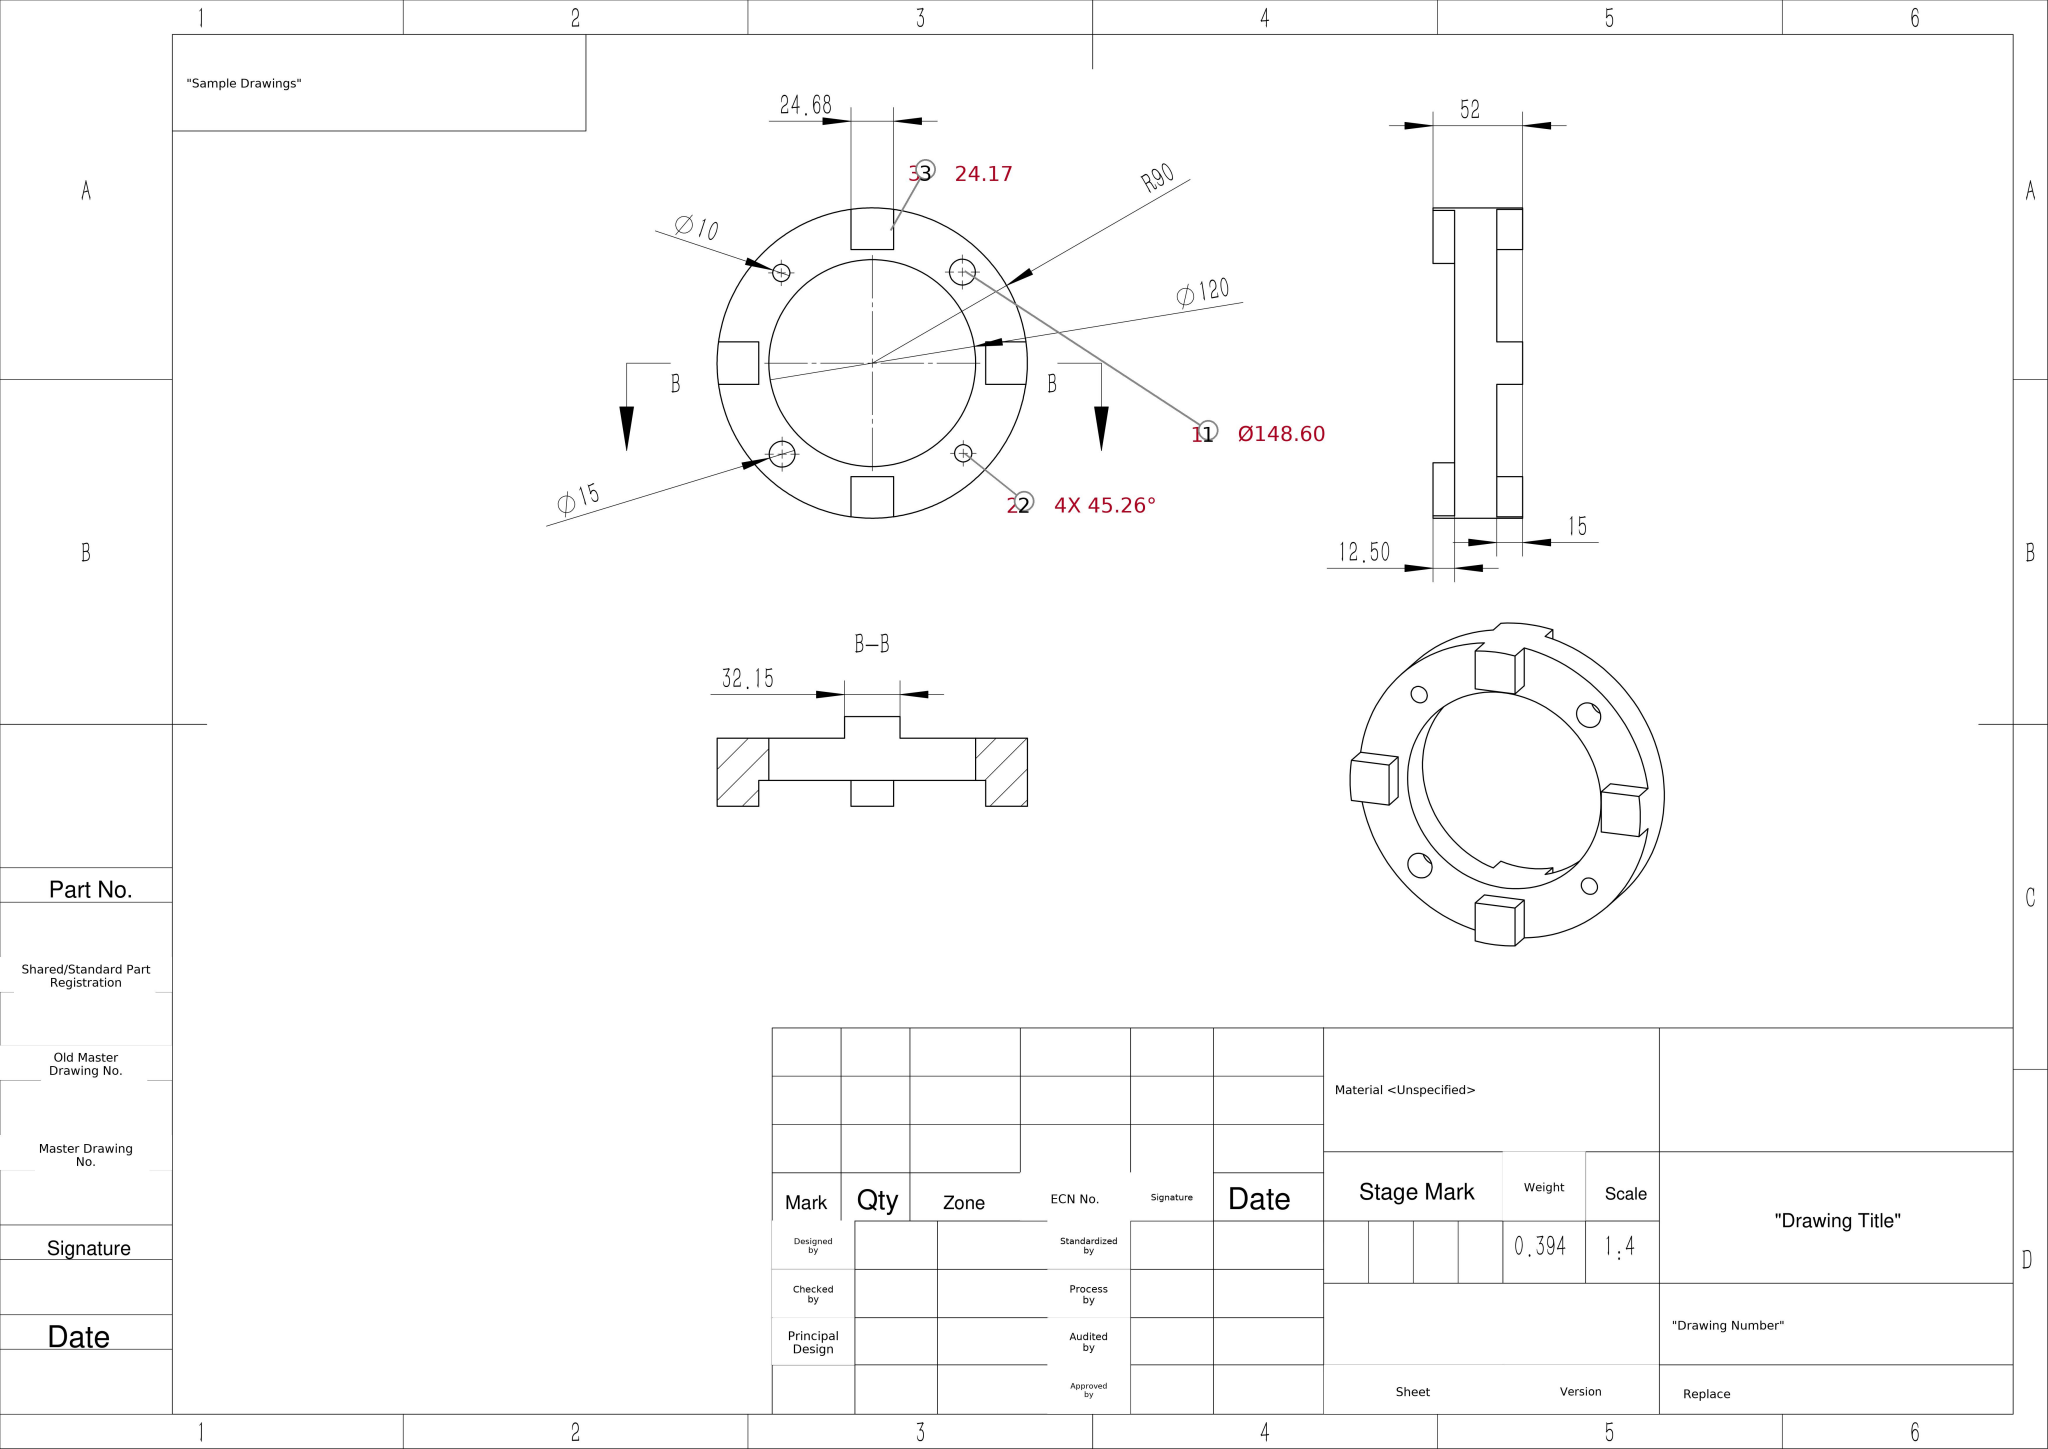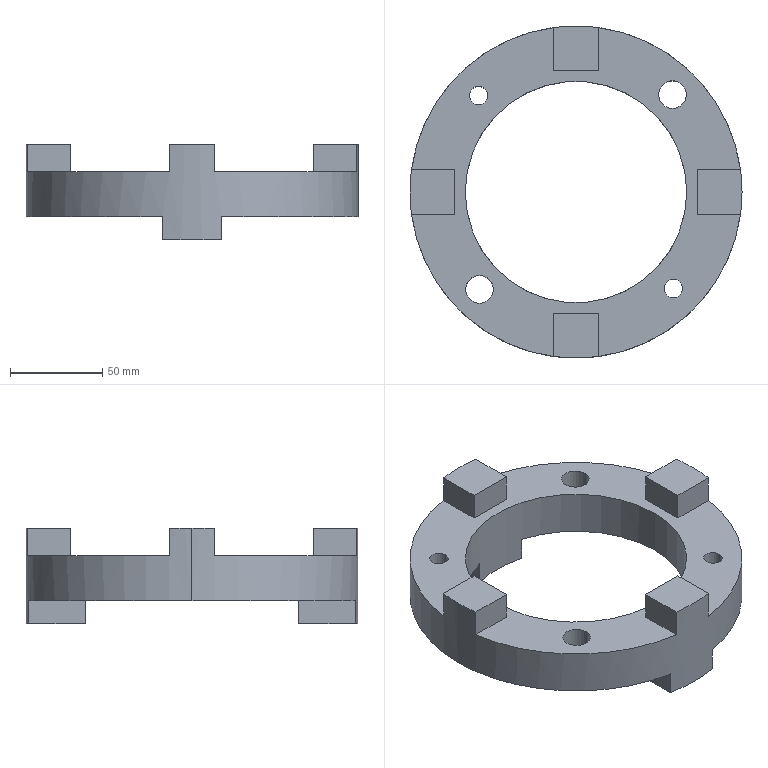Part | SolidWorks | mm | 1 solid | 37 faces | box 180 x 180 x 52 mm | volume 393536 mm3 | plane 25 | cylinder 12 | commonest cylinder face diameters 15 x4 10 x4 120 x2 180 x2
build123d program:
from build123d import *
from build123d.topology import SkipClean

# Parameters (mm, degrees)
SKETCH1_R           = 90
SKETCH1_R_2         = 60
BOSS_EXTRUDE1_DEPTH = 24.5
BOSS_EXTRUDE2_DEPTH = 15
BOSS_EXTRUDE3_START = 12.5
BOSS_EXTRUDE3_DEPTH = 12.5
SKETCH4_R           = 5
CUT_EXTRUDE1_DEPTH  = 84.5
SKETCH5_R           = 7.5
CUT_EXTRUDE2_DEPTH  = 84.5


with BuildPart() as part:
    # Sketch1 → Boss-Extrude1 (new body)
    with BuildSketch(Plane.XY):
        Circle(SKETCH1_R)
        Circle(SKETCH1_R_2, mode=Mode.SUBTRACT)
    extrude(amount=BOSS_EXTRUDE1_DEPTH)

    # Sketch2 → Boss-Extrude2 (add)
    with BuildSketch(Plane.XY.offset(24.5)):
        with BuildLine():
            Line((-65.831, 12.34), (-89.15, 12.34))
            ThreePointArc((-89.15, 12.34), (-90, 0), (-89.15, -12.34))
            Line((-89.15, -12.34), (-65.831, -12.34))
            Line((-65.831, -12.34), (-65.831, 12.34))
        make_face()
        with BuildLine():
            Line((-12.34, 65.831), (0, 65.831))
            Line((0, 65.831), (0, 90))
            ThreePointArc((0, 90), (-6.185, 89.787), (-12.34, 89.15))
            Line((-12.34, 89.15), (-12.34, 65.831))
        make_face()
        with BuildLine():
            Line((0, 90), (0, 65.831))
            Line((0, 65.831), (12.34, 65.831))
            Line((12.34, 65.831), (12.34, 89.15))
            ThreePointArc((12.34, 89.15), (6.185, 89.787), (0, 90))
        make_face()
        with BuildLine():
            ThreePointArc((90, 0), (89.787, 6.185), (89.15, 12.34))
            Line((89.15, 12.34), (65.831, 12.34))
            Line((65.831, 12.34), (65.831, -12.34))
            Line((65.831, -12.34), (89.15, -12.34))
            ThreePointArc((89.15, -12.34), (89.787, -6.185), (90, 0))
        make_face()
        with BuildLine():
            Line((-12.34, -65.831), (-12.34, -89.15))
            ThreePointArc((-12.34, -89.15), (0, -90), (12.34, -89.15))
            Line((12.34, -89.15), (12.34, -65.831))
            Line((12.34, -65.831), (-12.34, -65.831))
        make_face()
    extrude(amount=BOSS_EXTRUDE2_DEPTH)

    # Sketch3 → Boss-Extrude3 (add)
    with SkipClean():  # the faces are left unmerged after this step: merging them gives an invalid solid
        with BuildSketch(Plane(origin=(0, 0, 0), x_dir=(-1, 0, 0), z_dir=(0, 0, -1)).offset(BOSS_EXTRUDE3_START)):
            with BuildLine():
                ThreePointArc((16.077, -57.806), (0, -60), (-16.077, -57.806))
                Line((-16.077, -57.806), (-16.077, -88.552))
                ThreePointArc((-16.077, -88.552), (0, -90), (16.077, -88.552))
                Line((16.077, -88.552), (16.077, -57.806))
            make_face()
            with BuildLine():
                Line((0, 90), (0, 60))
                ThreePointArc((0, 60), (8.113, 59.449), (16.077, 57.806))
                Line((16.077, 57.806), (16.077, 88.552))
                ThreePointArc((16.077, 88.552), (8.071, 89.637), (0, 90))
            make_face()
            with BuildLine():
                ThreePointArc((-16.077, 57.806), (-8.113, 59.449), (0, 60))
                Line((0, 60), (0, 90))
                ThreePointArc((0, 90), (-8.071, 89.637), (-16.077, 88.552))
                Line((-16.077, 88.552), (-16.077, 57.806))
            make_face()
        extrude(amount=-BOSS_EXTRUDE3_DEPTH)

    # Sketch4 → Cut-Extrude1 (cut)
    with SkipClean():  # the faces are left unmerged after this step: merging them gives an invalid solid
        with BuildSketch(Plane.XY.offset(24.5)):
            with Locations((-52.778, 52.297)):
                Circle(SKETCH4_R)
            with Locations((52.778, -52.297)):
                Circle(SKETCH4_R)
        extrude(amount=-CUT_EXTRUDE1_DEPTH, mode=Mode.SUBTRACT)

    # Sketch5 → Cut-Extrude2 (cut)
    with SkipClean():  # the faces are left unmerged after this step: merging them gives an invalid solid
        with BuildSketch(Plane.XY.offset(24.5)):
            with Locations((52.297, 52.778)):
                Circle(SKETCH5_R)
            with Locations((-52.297, -52.778)):
                Circle(SKETCH5_R)
        extrude(amount=-CUT_EXTRUDE2_DEPTH, mode=Mode.SUBTRACT)


solid = part.part